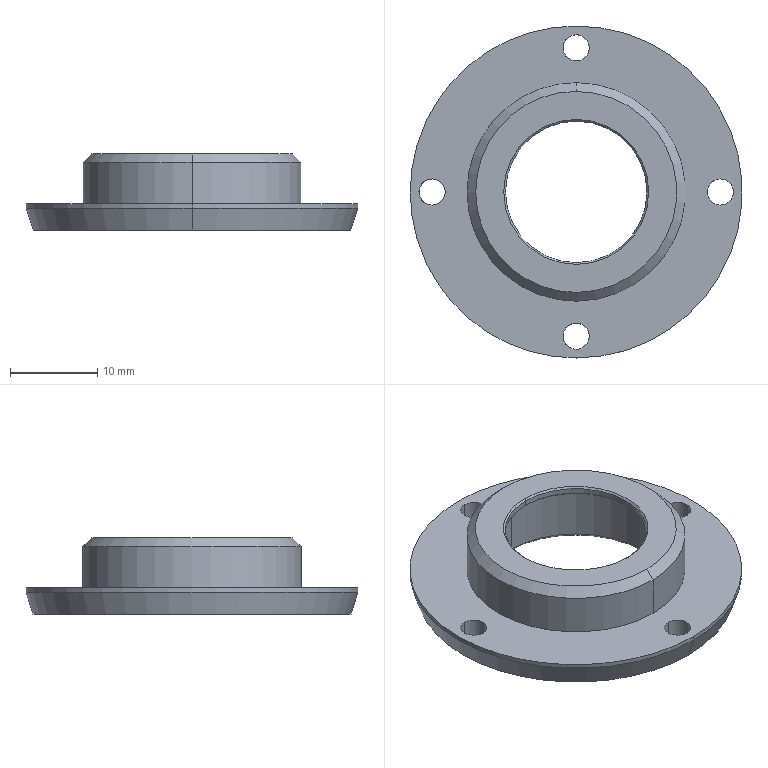CAM job | Mastercam | mm | 25 operations | part box 38 x 38 x 8.7
1. 3D High Speed (Area rest roughing) | 26 - 6 平铣刀
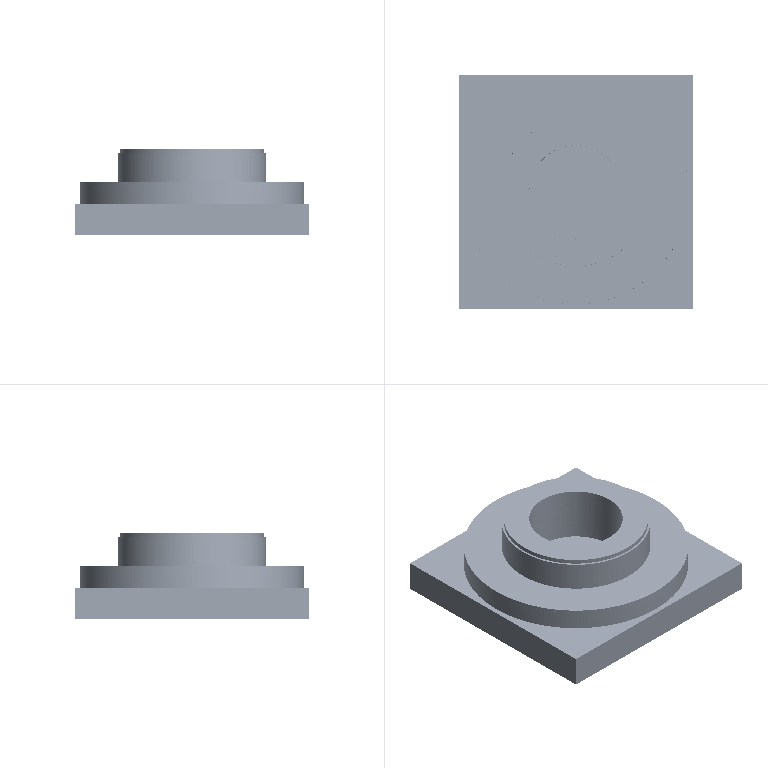2. Contour (2D) | 26 - 6 平铣刀
3. Contour (2D) | 26 - 6 平铣刀
4. Contour (2D) | 26 - 6 平铣刀
5. Contour (2D) | 26 - 6 平铣刀
6. Model Chamfer | 11 - 4 倒角刀
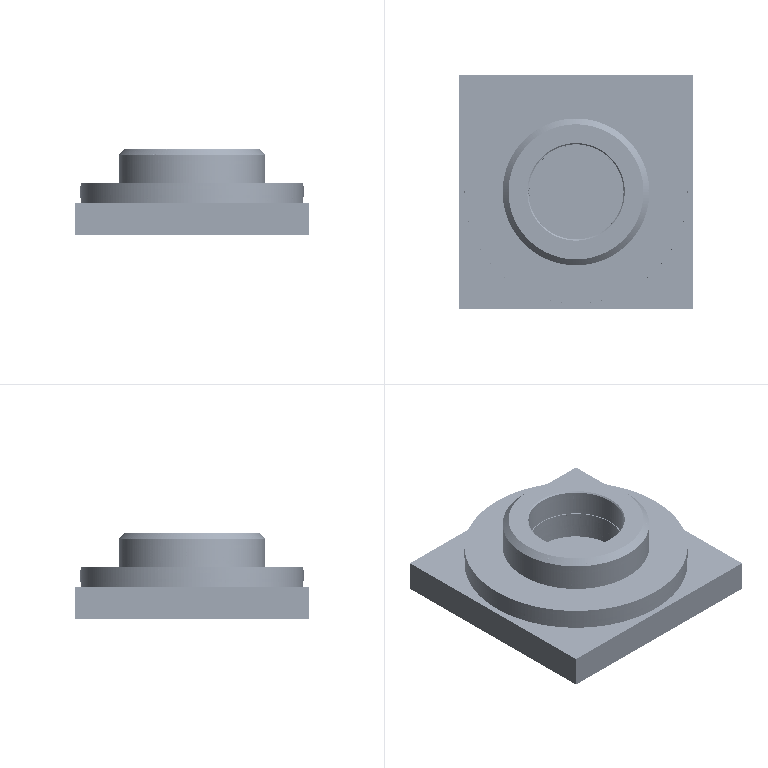7. Model Chamfer | 11 - 4 倒角刀
8. Facing | 2 - 10C
9. Facing | 3 - 10J
10. 3D High Speed (Area rest roughing) | 4 - 4C
11. Contour (2D) | 5 - 4J
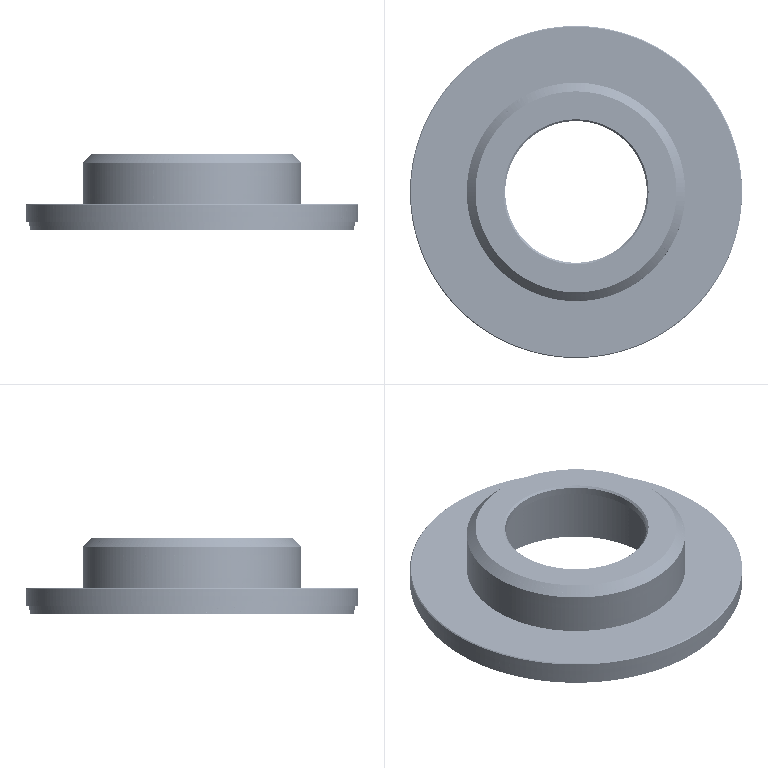12. Contour (Ramp) | 12 - 2C
13. Contour (2D) | 13 - 2J
14. 3D High Speed (Waterline rest passes) | 16 - 1.5 平铣刀
15. Pocket (Standard) | 16 - 1.5 平铣刀
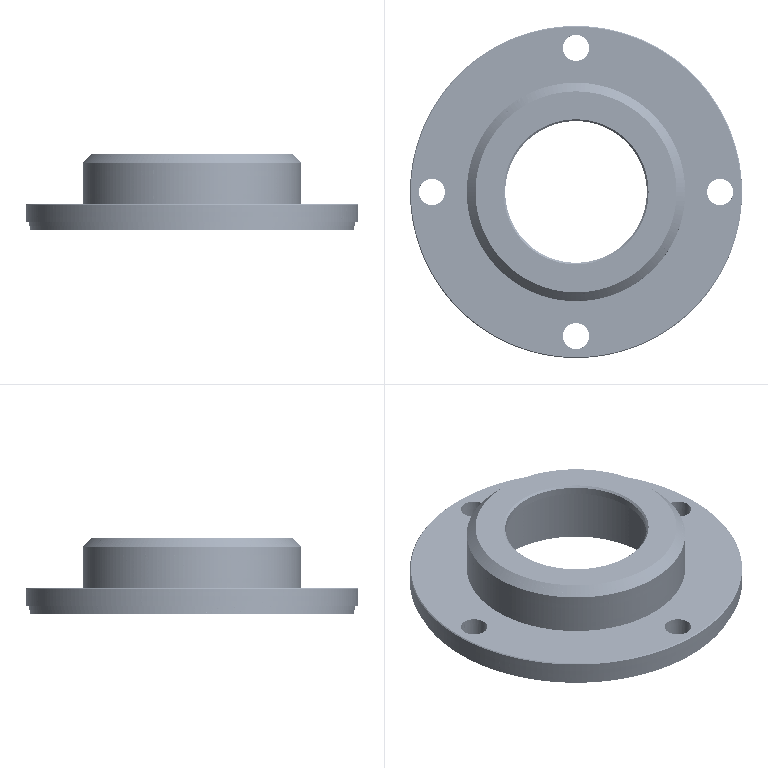16. Pocket (Standard) | 16 - 1.5 平铣刀
17. Contour (2D) | 31 - 10 槽铣刀或锯式刀具
18. Thread Mill | 32 - 2.4 螺纹铣刀
19. Chamfer Drill | 11 - 4 倒角刀
20. Model Chamfer | 11 - 4 倒角刀
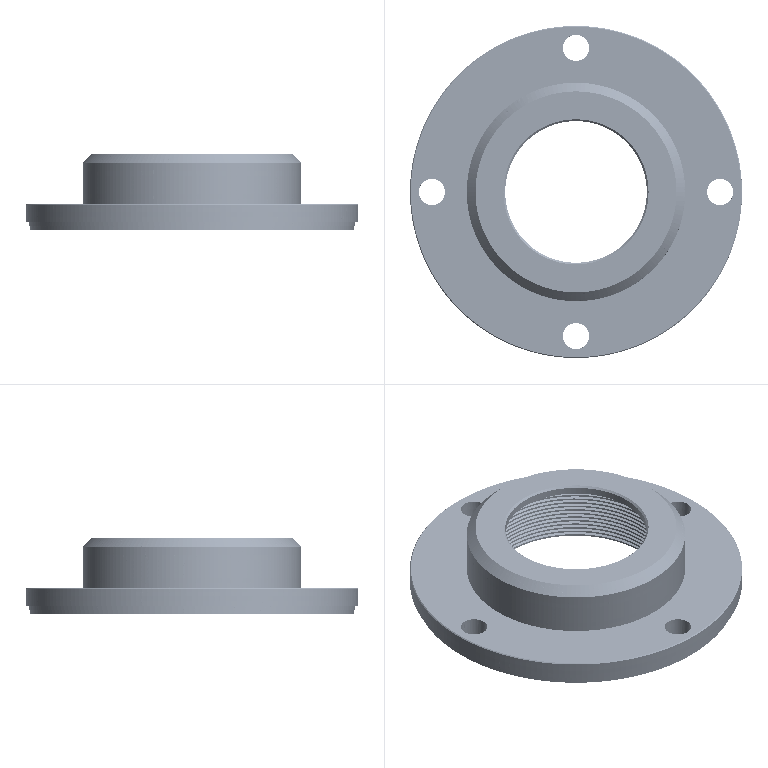21. Model Chamfer | 11 - 4 倒角刀
22. Surface Finish Flowline | 15 - 4 圆鼻铣刀
23. Contour (Ramp) | 2 - 10C
24. Contour (2D) | 3 - 10J
25. Contour (2D chamfer) | 6 - 6 倒角刀